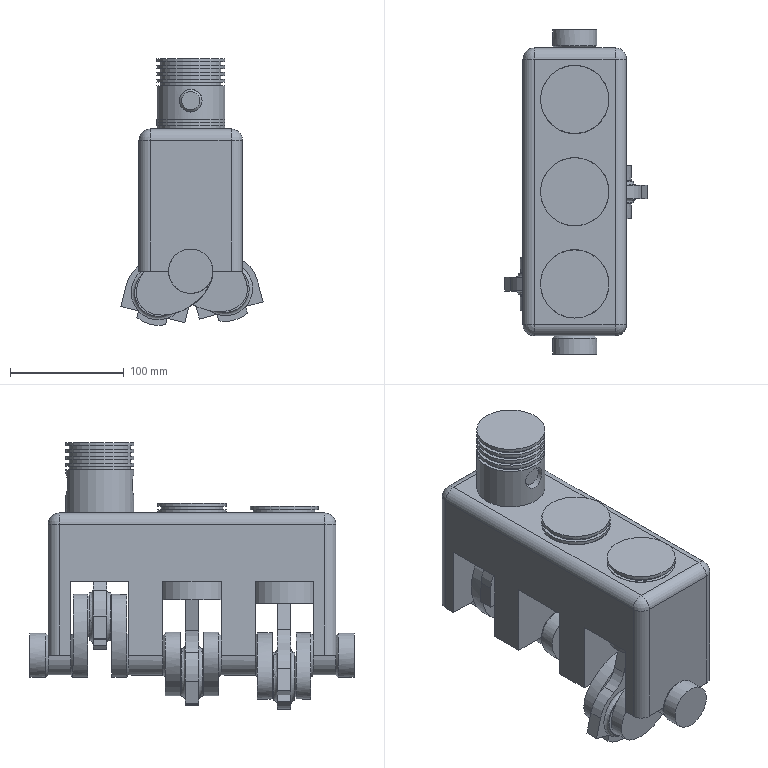Assembly | NX | mm | 11 component files | 38 solids | 329 faces | box 125.03 x 285 x 234.63 mm | volume 2309172 mm3 | plane 158 | cylinder 129 | cone 20 | torus 12 | other 6 | sphere 4 | commonest cylinder face diameters 20 x26 48 x21 60 x15 54 x12 35 x11 58 x9 44 x6 42 x6
Bill of materials:
unnamed part 1 | 1 |  | Rectangular block with rounded edges. Three round holes in a row go down through the top face. The underside is cut away into three slots under the holes, which leaves short legs between and at the ends of the block.
unnamed part 2 | 3 |  | Solid-looking cylinder with a flat top. Five evenly spaced ring grooves run around it near the top. One round hole goes straight across through the body below the grooves, with shallow scooped areas on the outside around each end of the hole. Overall it looks like a piston.
unnamed part 3 | 3 |  | Plain solid round pin with chamfered edges at both ends. Its length is about 2.5 to 3 times its diameter.
unnamed part 4 | 3 |  | Long link with a small round eye at one end, a straight narrow beam, and a wider end with a larger round bore. Around the large bore there is a raised ring, and below it a flat edge with a small curved tab. Overall it looks like a connecting rod.
unnamed part 5 | 1 |  | Stepped shaft with journals sharing one centre line, joined by disc-shaped webs to three offset cylindrical pins. Seen end-on, the webs form three lobes spread around the axis. Overall it looks like a three-throw crankshaft.
Mates:
1. fix | housing 1 component
2. touch align | crankshaft 1 face | housing 1 face
3. center | crankshaft 1 face | crankshaft 1 face | housing 1 face | housing 1 face
4. touch align | piston_rod 3 face | crankshaft 1 face
5. center | piston_rod 3 face | piston_rod 3 face | crankshaft 1 face | crankshaft 1 face
6. touch align | piston 3 face | piston_rod 3 face
7. center | piston_rod 3 face | piston_rod 3 face | piston 3 face
8. touch align | piston_pin 3 face | piston 3 face
9. center | piston_pin 3 face | piston_pin 3 face | piston 3 face
10. touch align | piston 3 face | housing 1 face
11. touch align | piston 2 face | piston_rod 2 face
12. center | piston_rod 2 face | piston_rod 2 face | piston 2 face
13. touch align | crankshaft 1 face | piston_rod 2 face
14. distance | piston 2 face | housing 1 face
15. touch align | piston_pin 2 face | piston 2 face
16. center | piston_pin 2 face | piston_pin 2 face | piston 2 face
17. touch align | piston_rod 1 face | crankshaft 1 face
18. center | crankshaft 1 face | crankshaft 1 face | piston_rod 1 face | piston_rod 1 face
19. touch align | piston 1 face | piston_rod 1 face
20. center | piston_rod 1 face | piston_rod 1 face | piston 1 face
21. distance | piston 1 face | housing 1 face
22. touch align | piston_pin 1 face | piston 1 face
23. center | piston_pin 1 face | piston_pin 1 face | piston 1 face